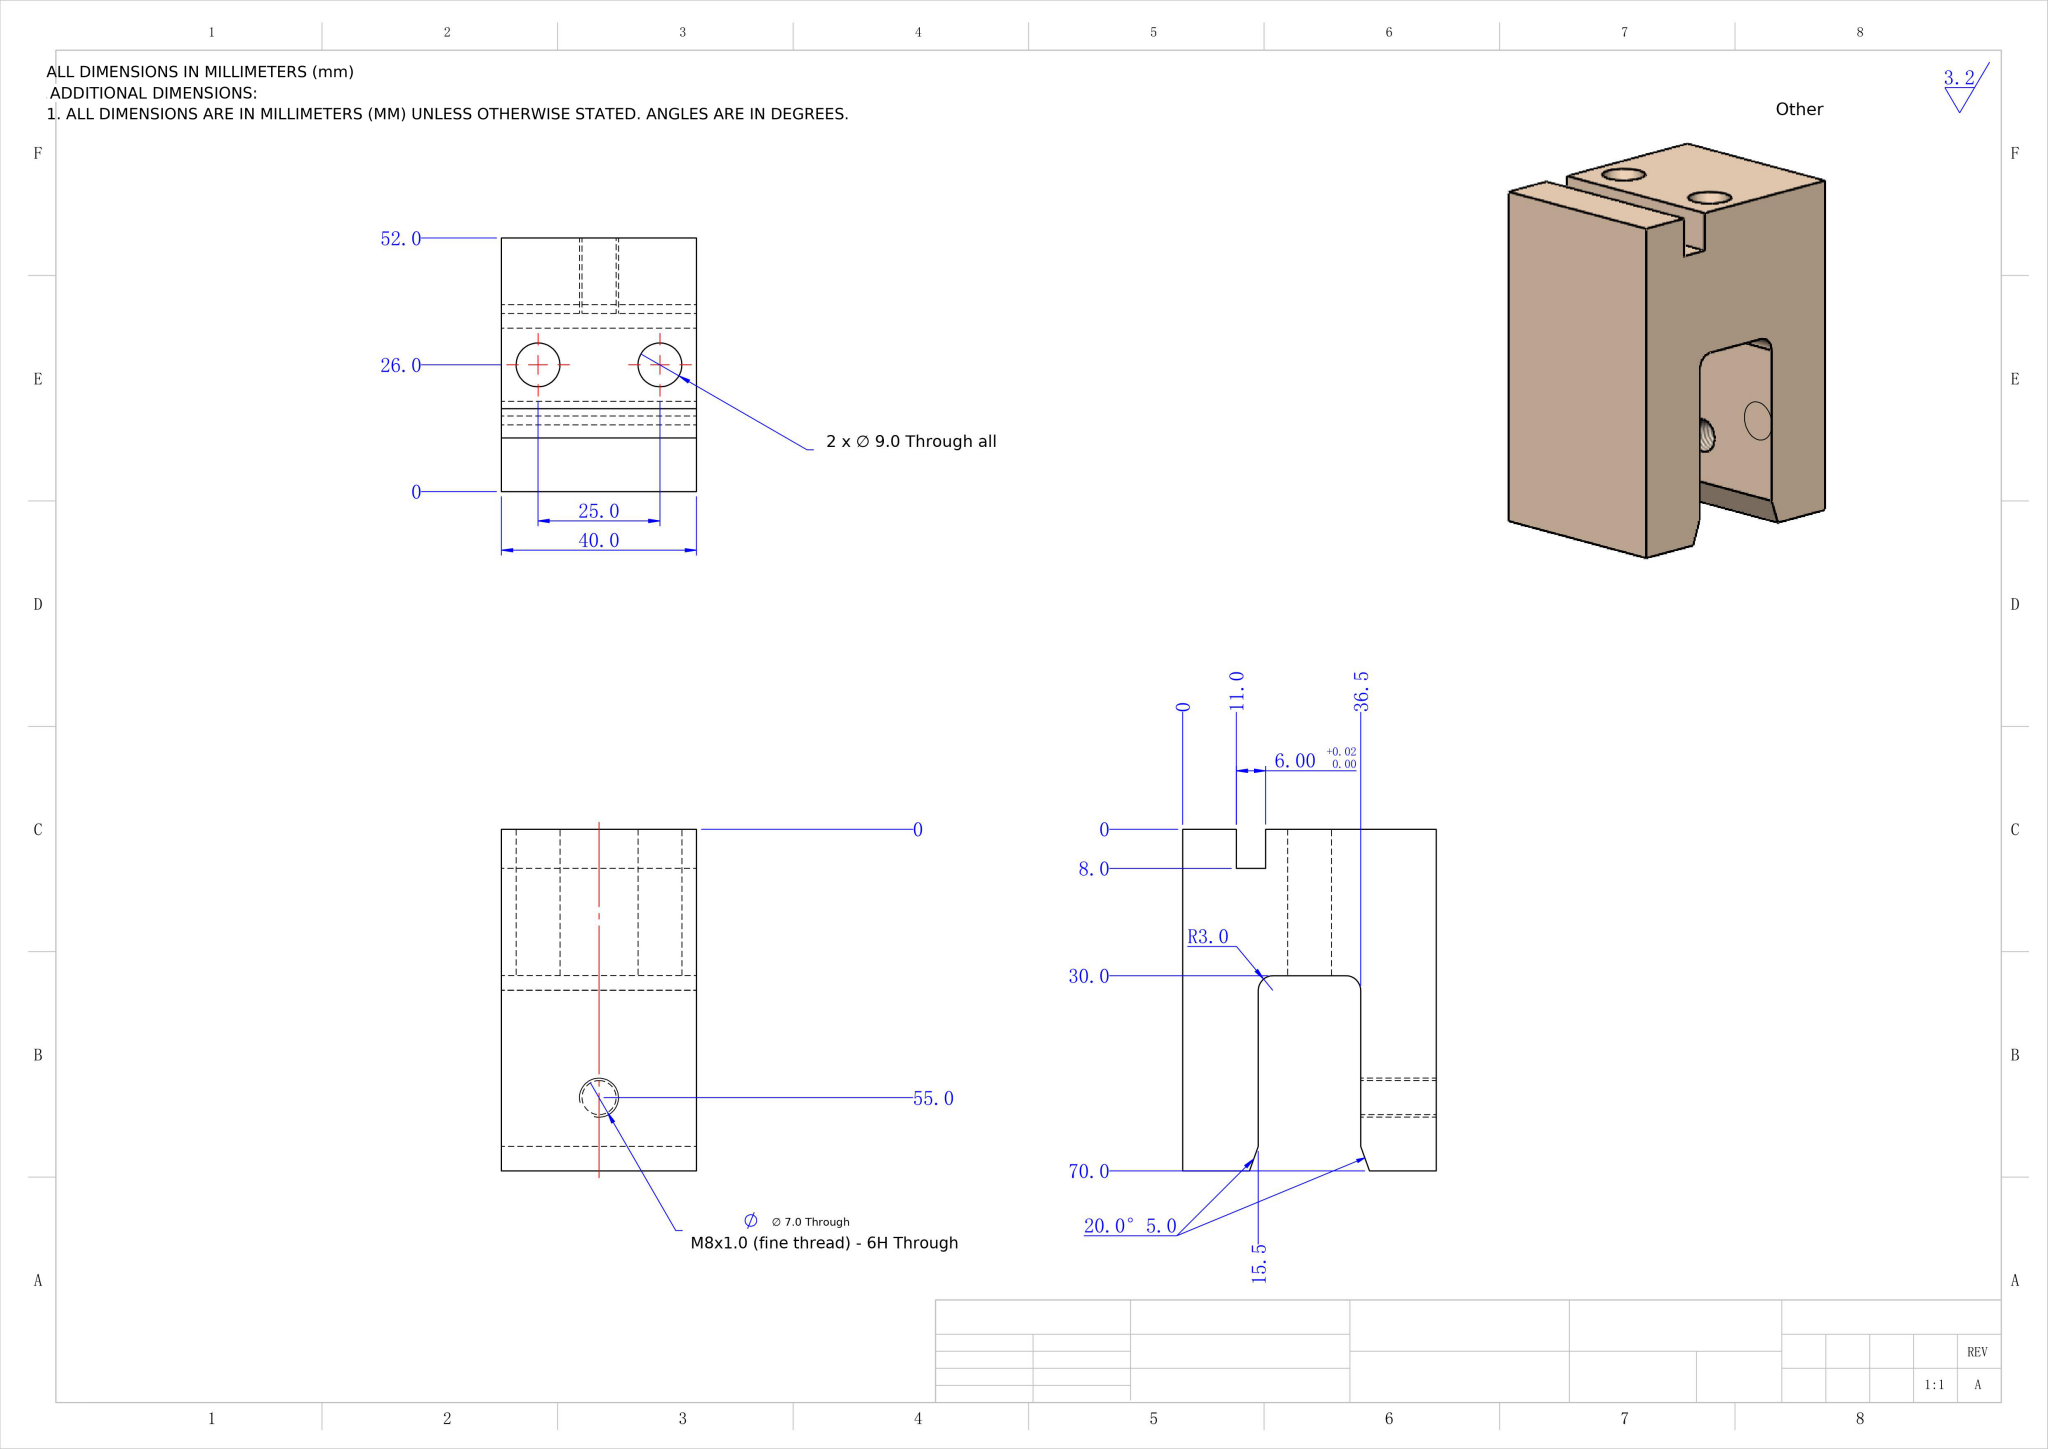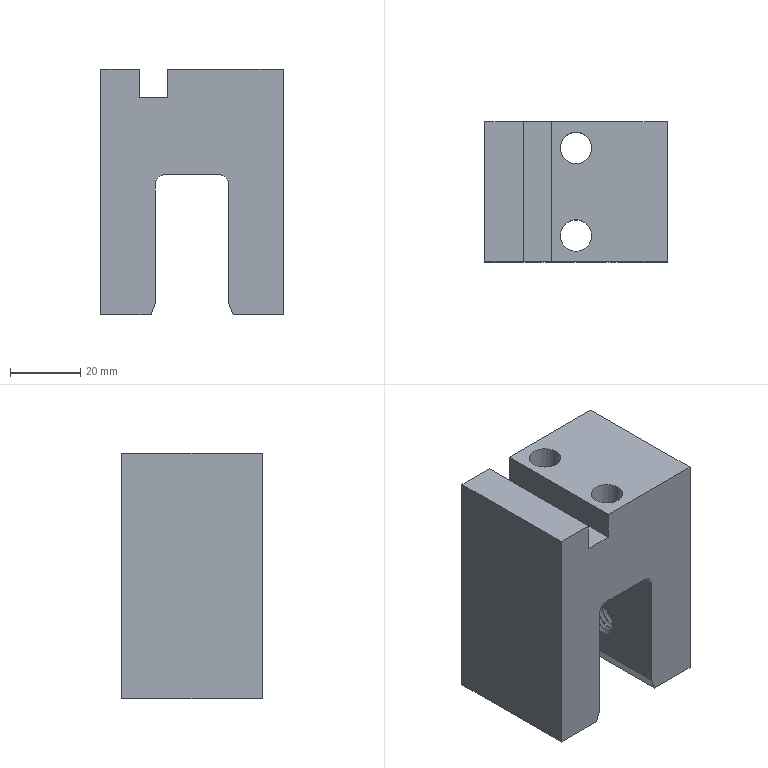Part | NX | mm | Stepped Dual-Platform Bore Mounting Block | 1 solid | 34 faces | box 52 x 40 x 70 mm | volume 104649 mm3 | plane 17 | cylinder 15 | spline 2 | commonest cylinder face diameters 8 x10 6 x2 9 x2 10 x1